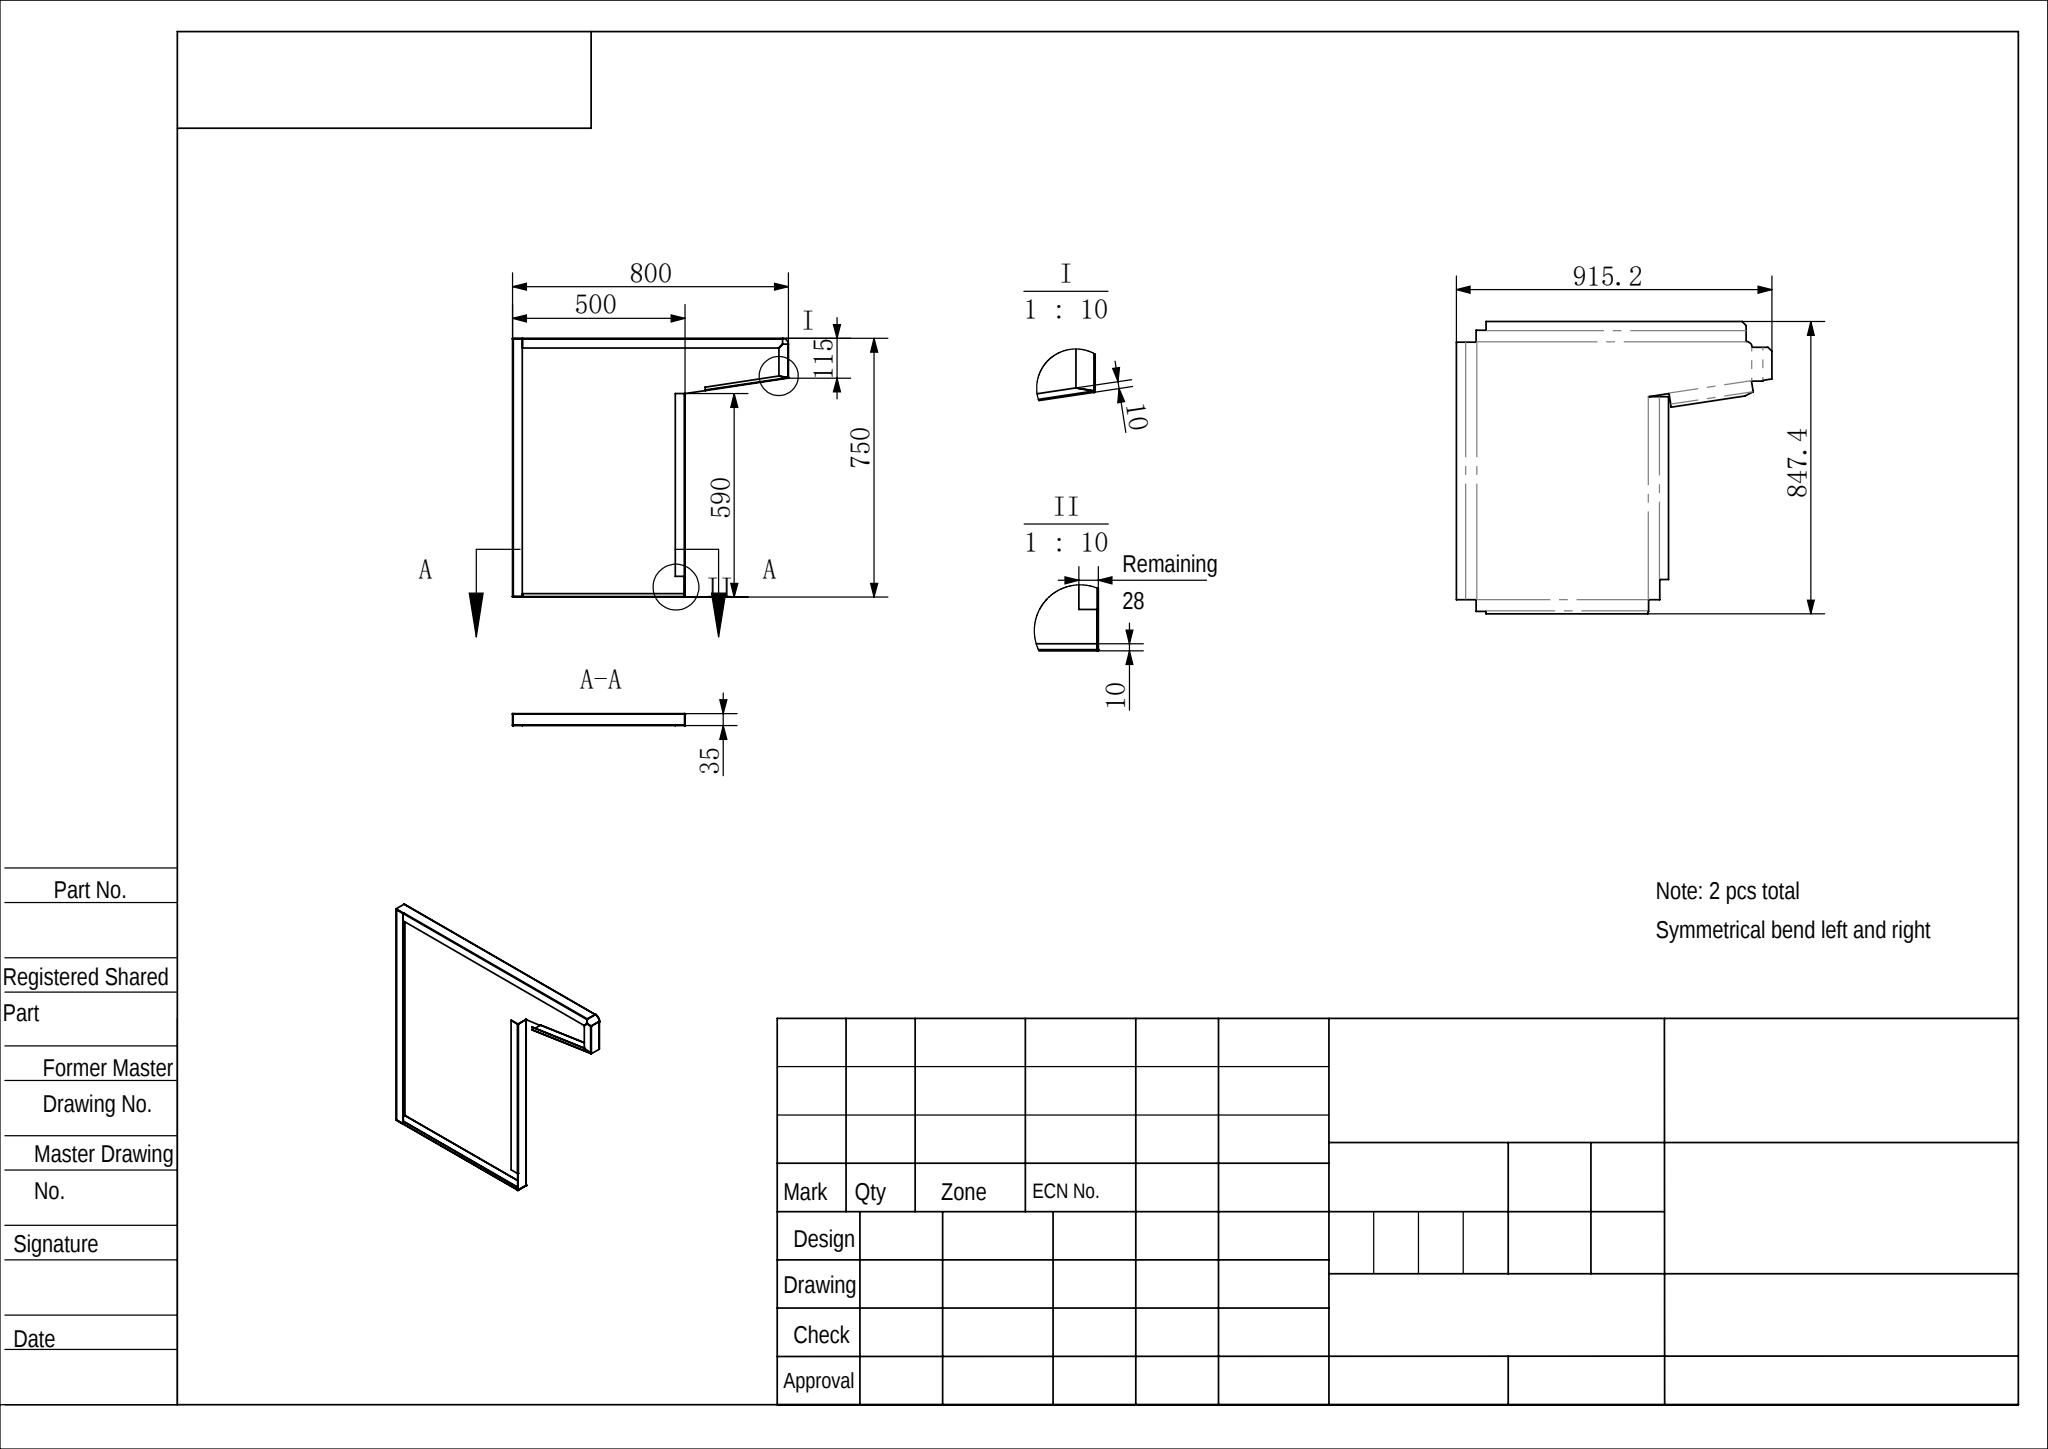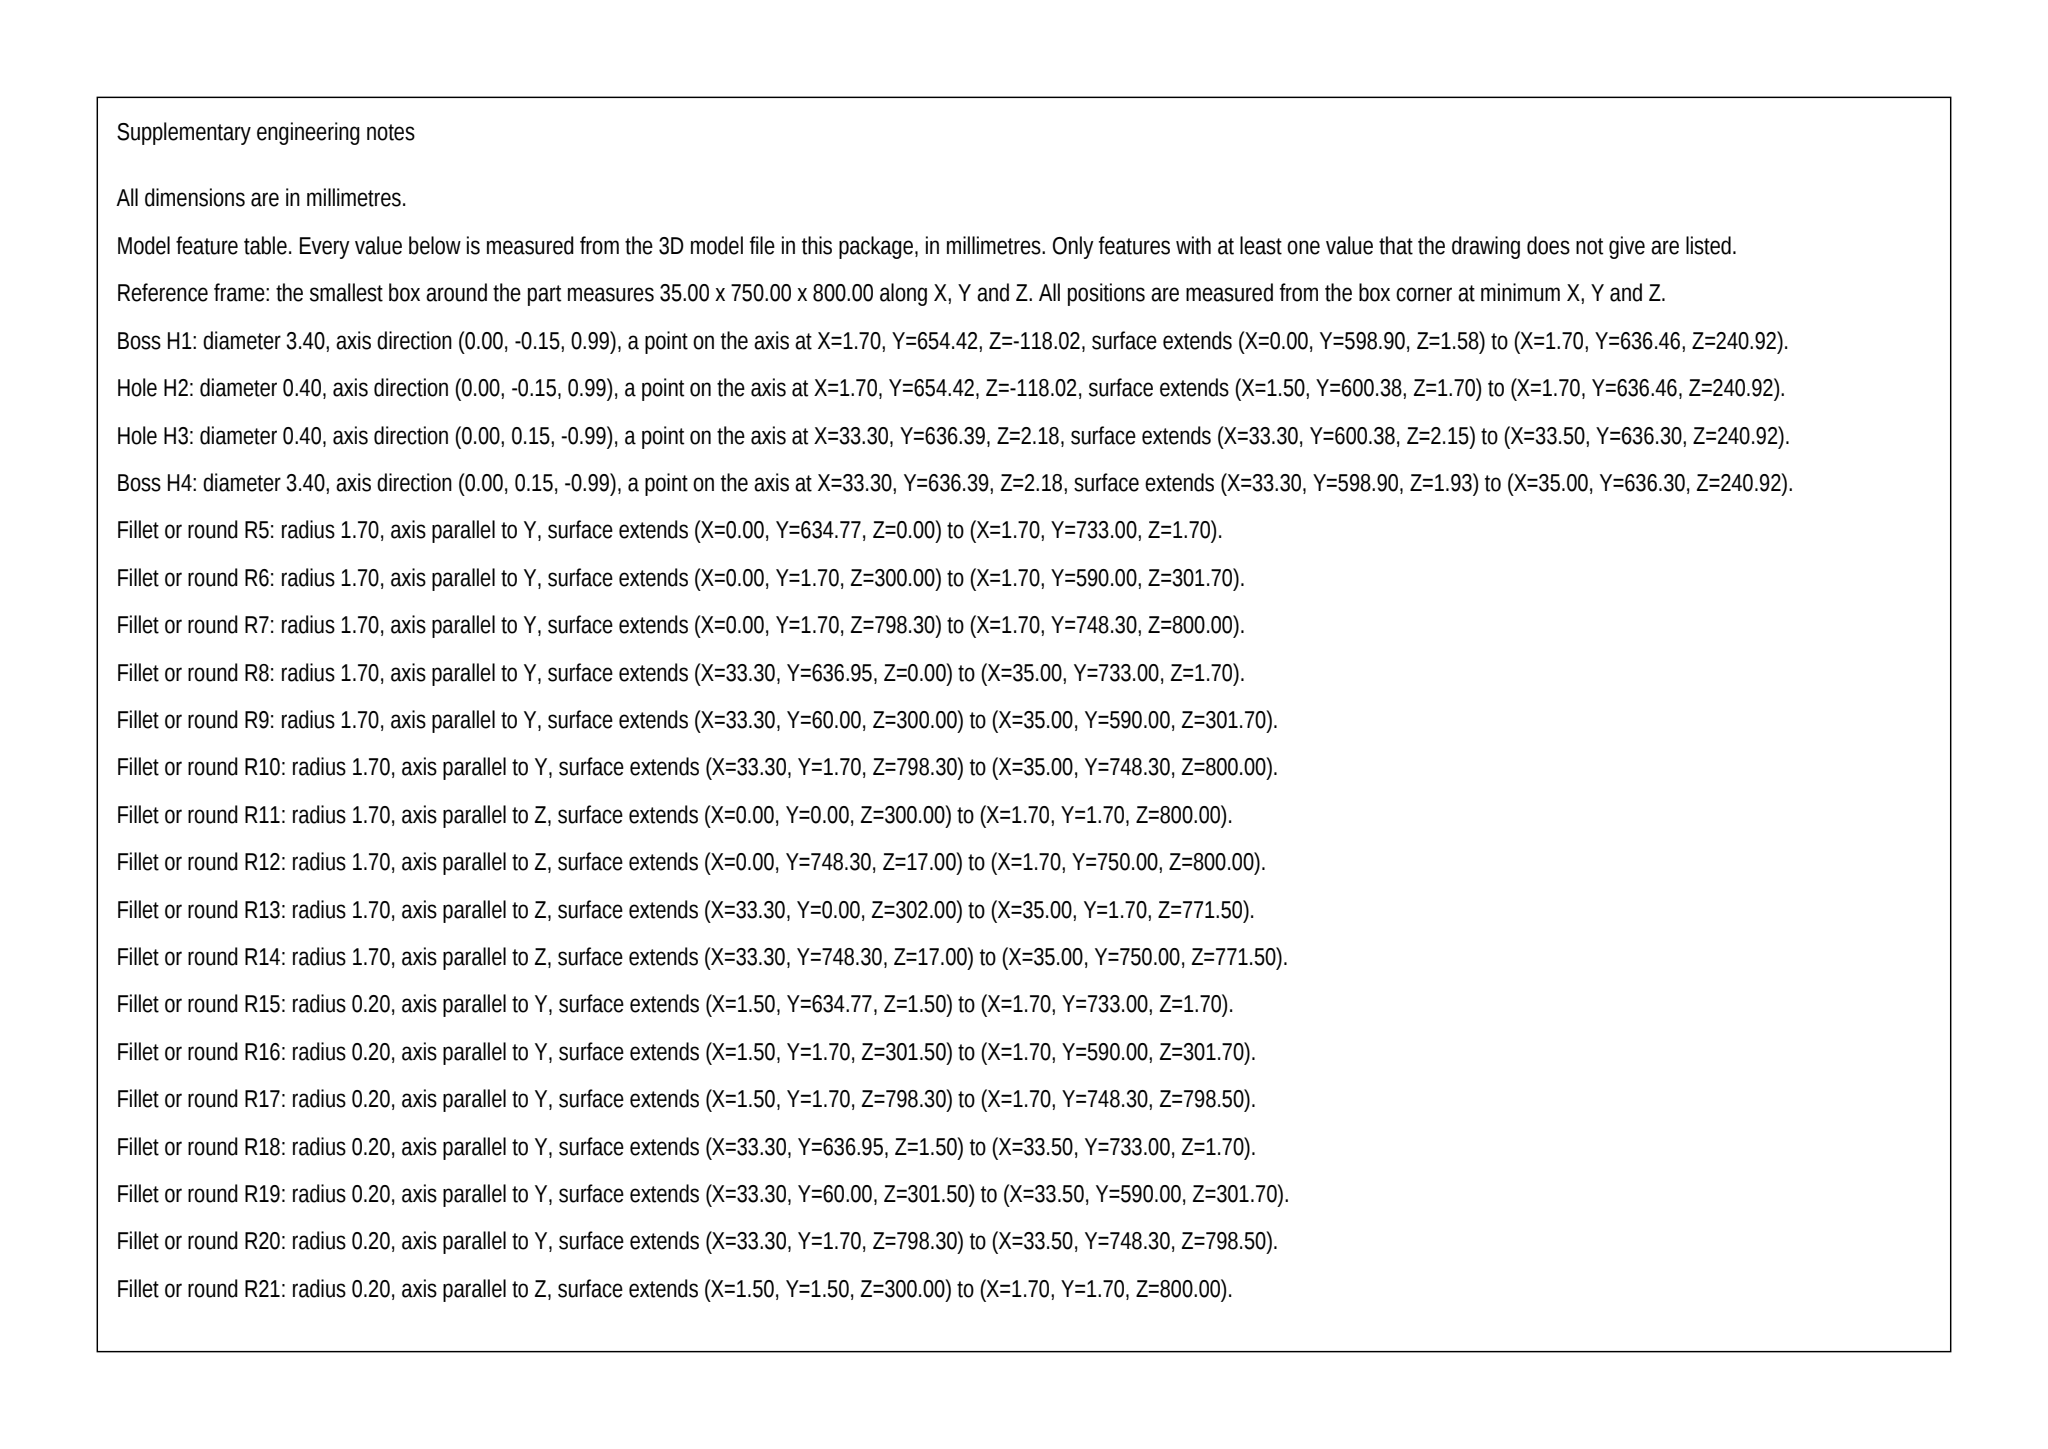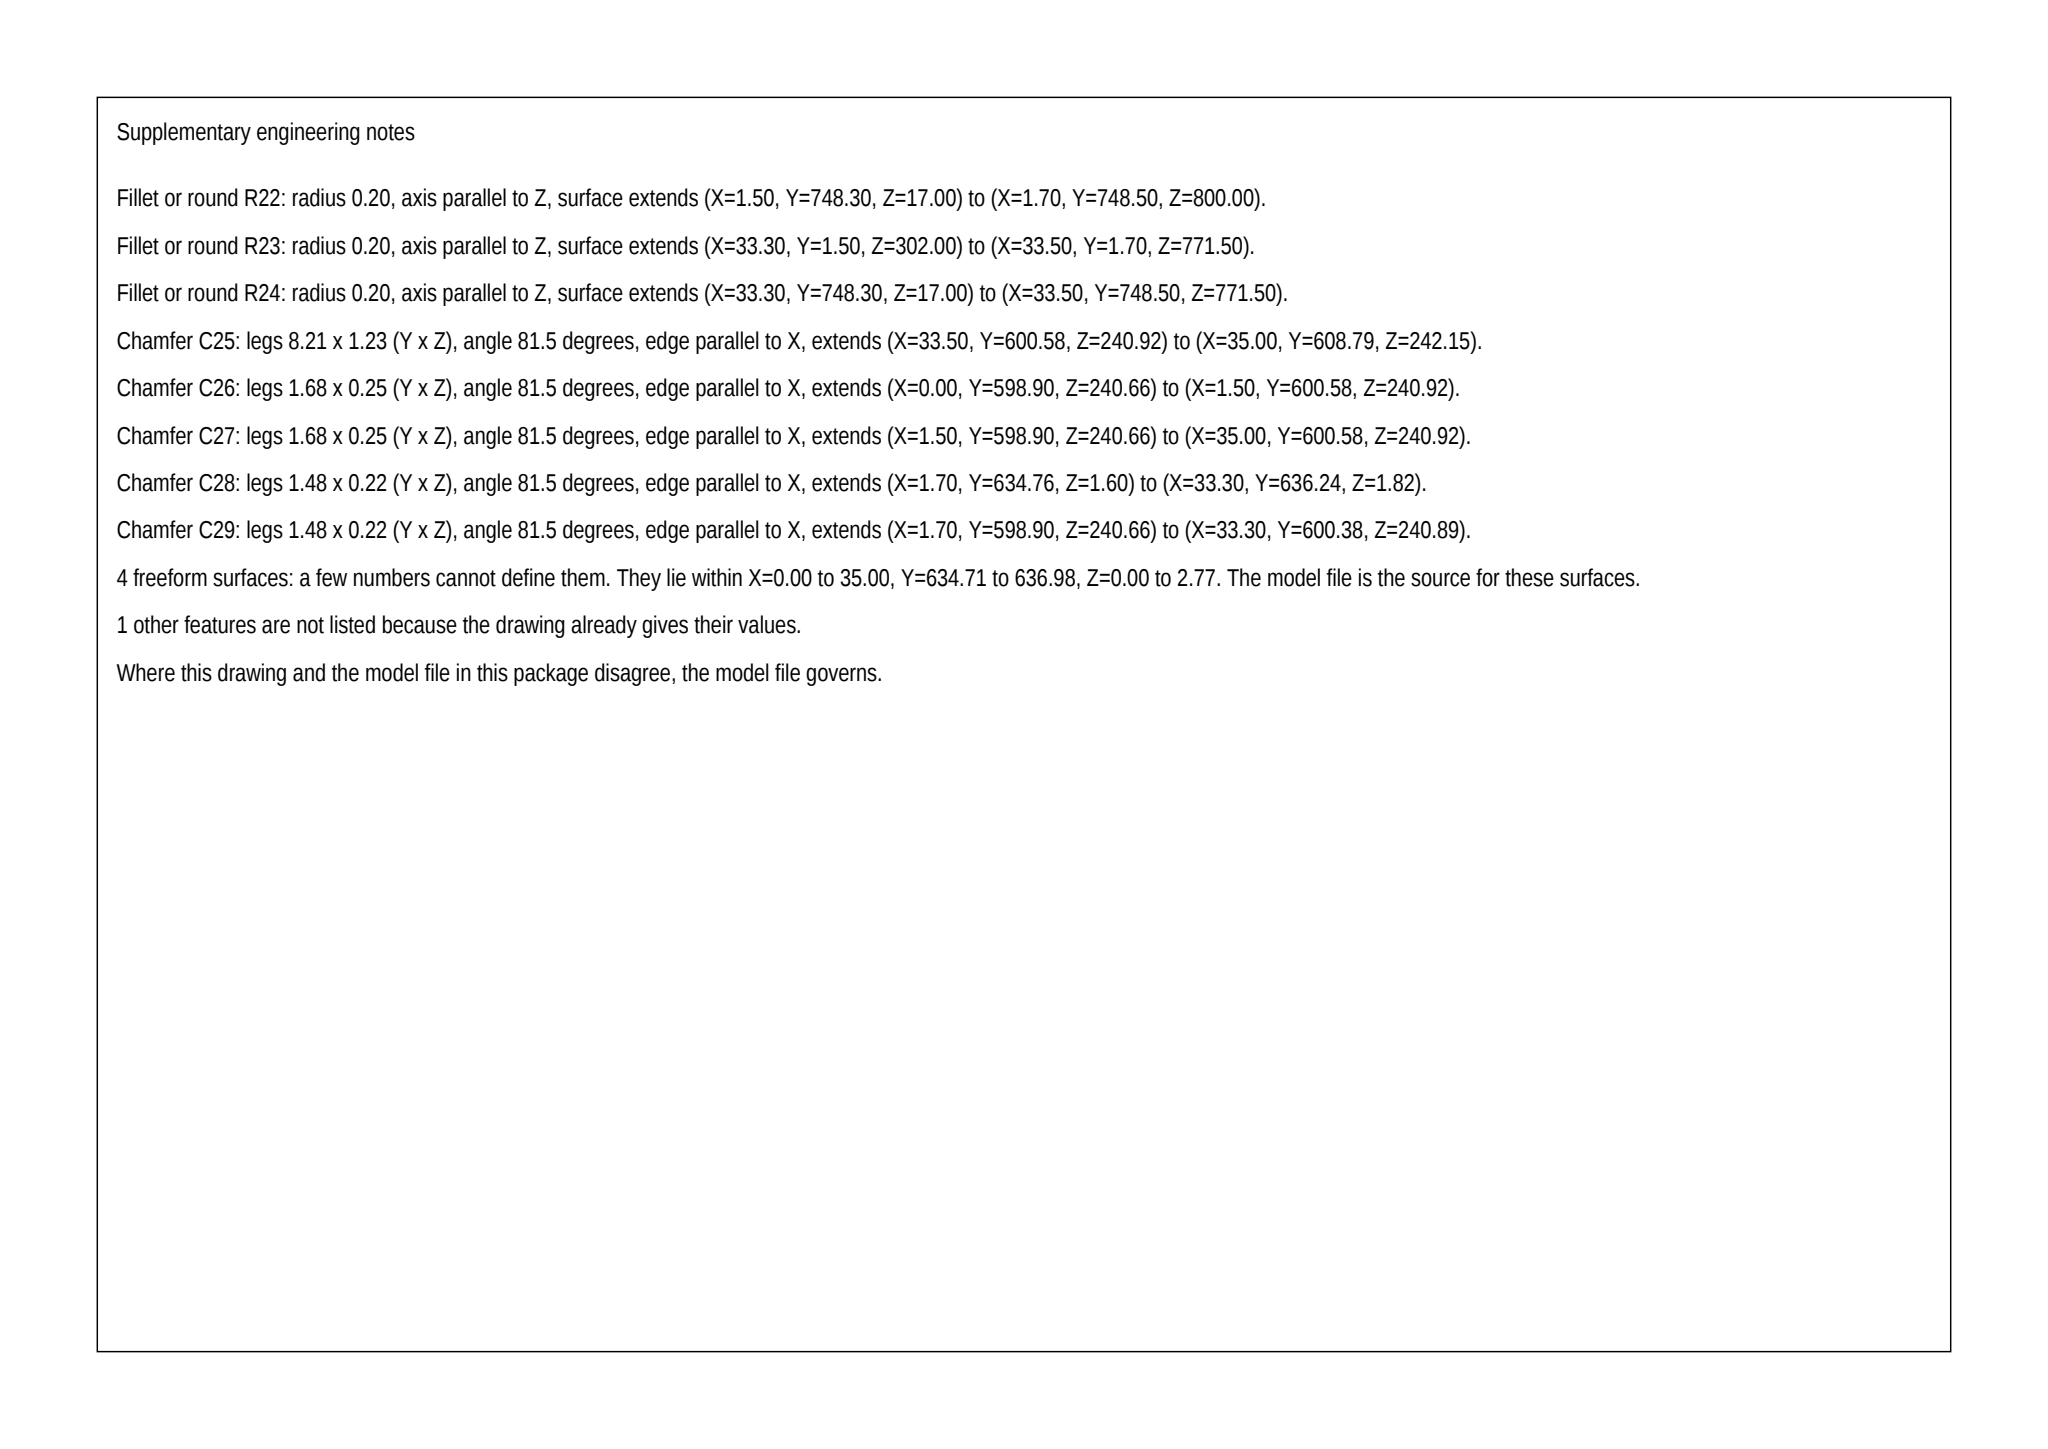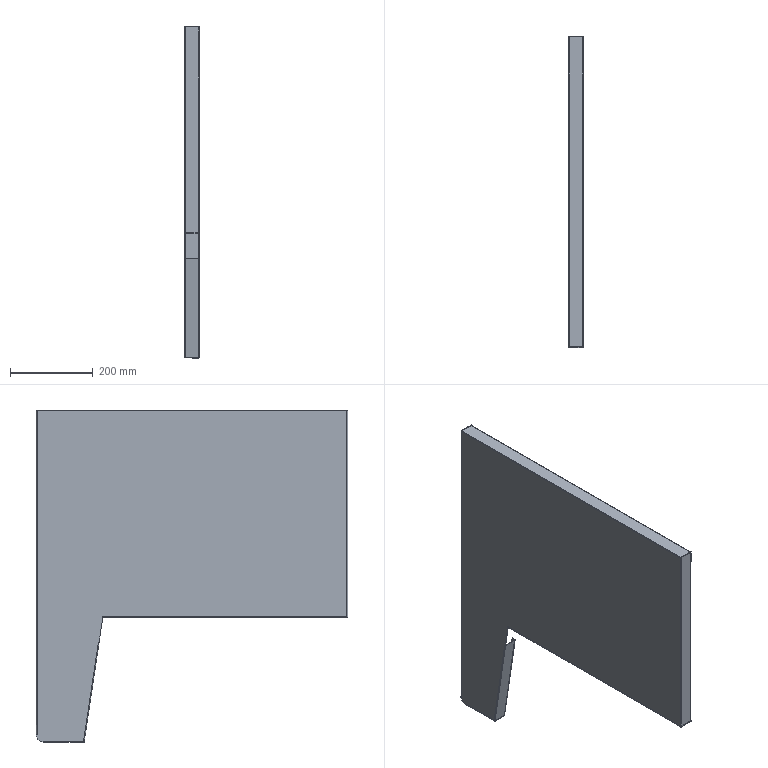Part | SolidWorks | mm | 1 solid | 125 faces | box 35 x 750 x 800 mm | volume 862500 mm3 | plane 96 | cylinder 25 | spline 4 | commonest cylinder face diameters 3.4 x12 0.4 x12 34 x1
Drawing notes:
35 FLG x 1.5 SKIN TYP ALL EDGES INCL SLOPE & NOTCH; ALL FLGS BENT TO SAME SIDE | from the solid: bbox x=35.03; skin planes x=33.52/35.02 (1.5 thk); all bend cyl axes at x=1.72/33.32 on bot, top, end, notch and sloped edges; flange material to x=0.02
ALL BENDS 90°, INSIDE R0.2, OUTSIDE R1.7 | from the solid: Coaxial cyls dia 0.4 & 3.4 at x=1.72/33.32, y=1.7/748.3, z=1.72/798.32; mating faces mutually perpendicular planes (x=0.02/1.52/33.52/35.02, y=0.0/1.5/748.5/750.0, z=0.02/1.52/798.52/800.02)
SLOPE BREAK 235 FROM 500 LINE, RISE 45; 65 FLAT TO 115 END EDGE | from the solid: notch line z=300.02/302.02 (500 from z=800 edge); slope y=590 to y=634.78 (=750-115); slanted bend len 239.25 = sqrt(235^2+45^2); flat run 65 to end edge z=0
TOP CNR AT 115 END EDGE: R17 OUTSIDE RND, CTR 17 FROM BOTH EDGES | from the solid: cyl dia 34 axis x at y=733.0, z=17.02, len 1.5 (skin); tangent planes z=17.02 (x5) and y=733.0 (x5); top edge bend len 783.0 = 800.02-17.02
DET II: 28 WIDE FROM 500 LINE x 10 UP FROM BOT EDGE | from the solid: Planes z=300.02 and z=328.02 => 28 remaining; plane y=10.0 vs bottom edge y=0.0 => 10; inner member faces z=300.02/302.02 = drawing 500 line
DET I: SKIN FOLD 10 WIDE x 239.3 LG, FULL SLOPED EDGE 590 PT TO SLOPE BREAK | from the solid: Sloped bend cyls dia 0.4/3.4 axis z at [x1.72,y654.42] L=239.25/239.47 and [x33.32,y636.39] L=238.76/238.99, between y=590 and y=634.78; fold return 10 per plane y=634.78
TOP FLG BEND LINE 754.5 LG; 28.5 CNR RELIEF AT LH END EDGE | from the solid: Z-axis bend cyl at x=33.32,y=748.3 L=754.5 (z 17.02-771.52) vs outer x=1.72,y=748.3 L=783.0 to z=800.02; planes z=771.52 x6 = 28.5 from z=800.02
BOT FLG BEND LINE 469.5 LG; 28.5 RELIEF LH END, 2 AT 500 LINE | from the solid: Z-axis bend cyl at x=33.32,y=1.7 L=469.5 (z 302.02-771.52) vs outer x=1.72,y=1.7 L=500.0 (z 300.02-800.02)
500-LINE FLG BEND LINE 530 LG; STARTS 60 UP FROM BOT EDGE | from the solid: Y-axis bend cyl at x=33.32,z=301.72 L=530.0 with y planes 60.0 (x3) and 590.0; outer x=1.72,z=301.72 L=588.3 from y=1.7
SLOPED FLG BEND LINE 238.8 LG; NO CNR RELIEF AT 590 PT OR 65 FLAT | from the solid: Sloped bend cyl x=33.32 L=238.76/238.99 vs outer x=1.72 L=239.25; ends at y=590 cnr and y=634.78 flat